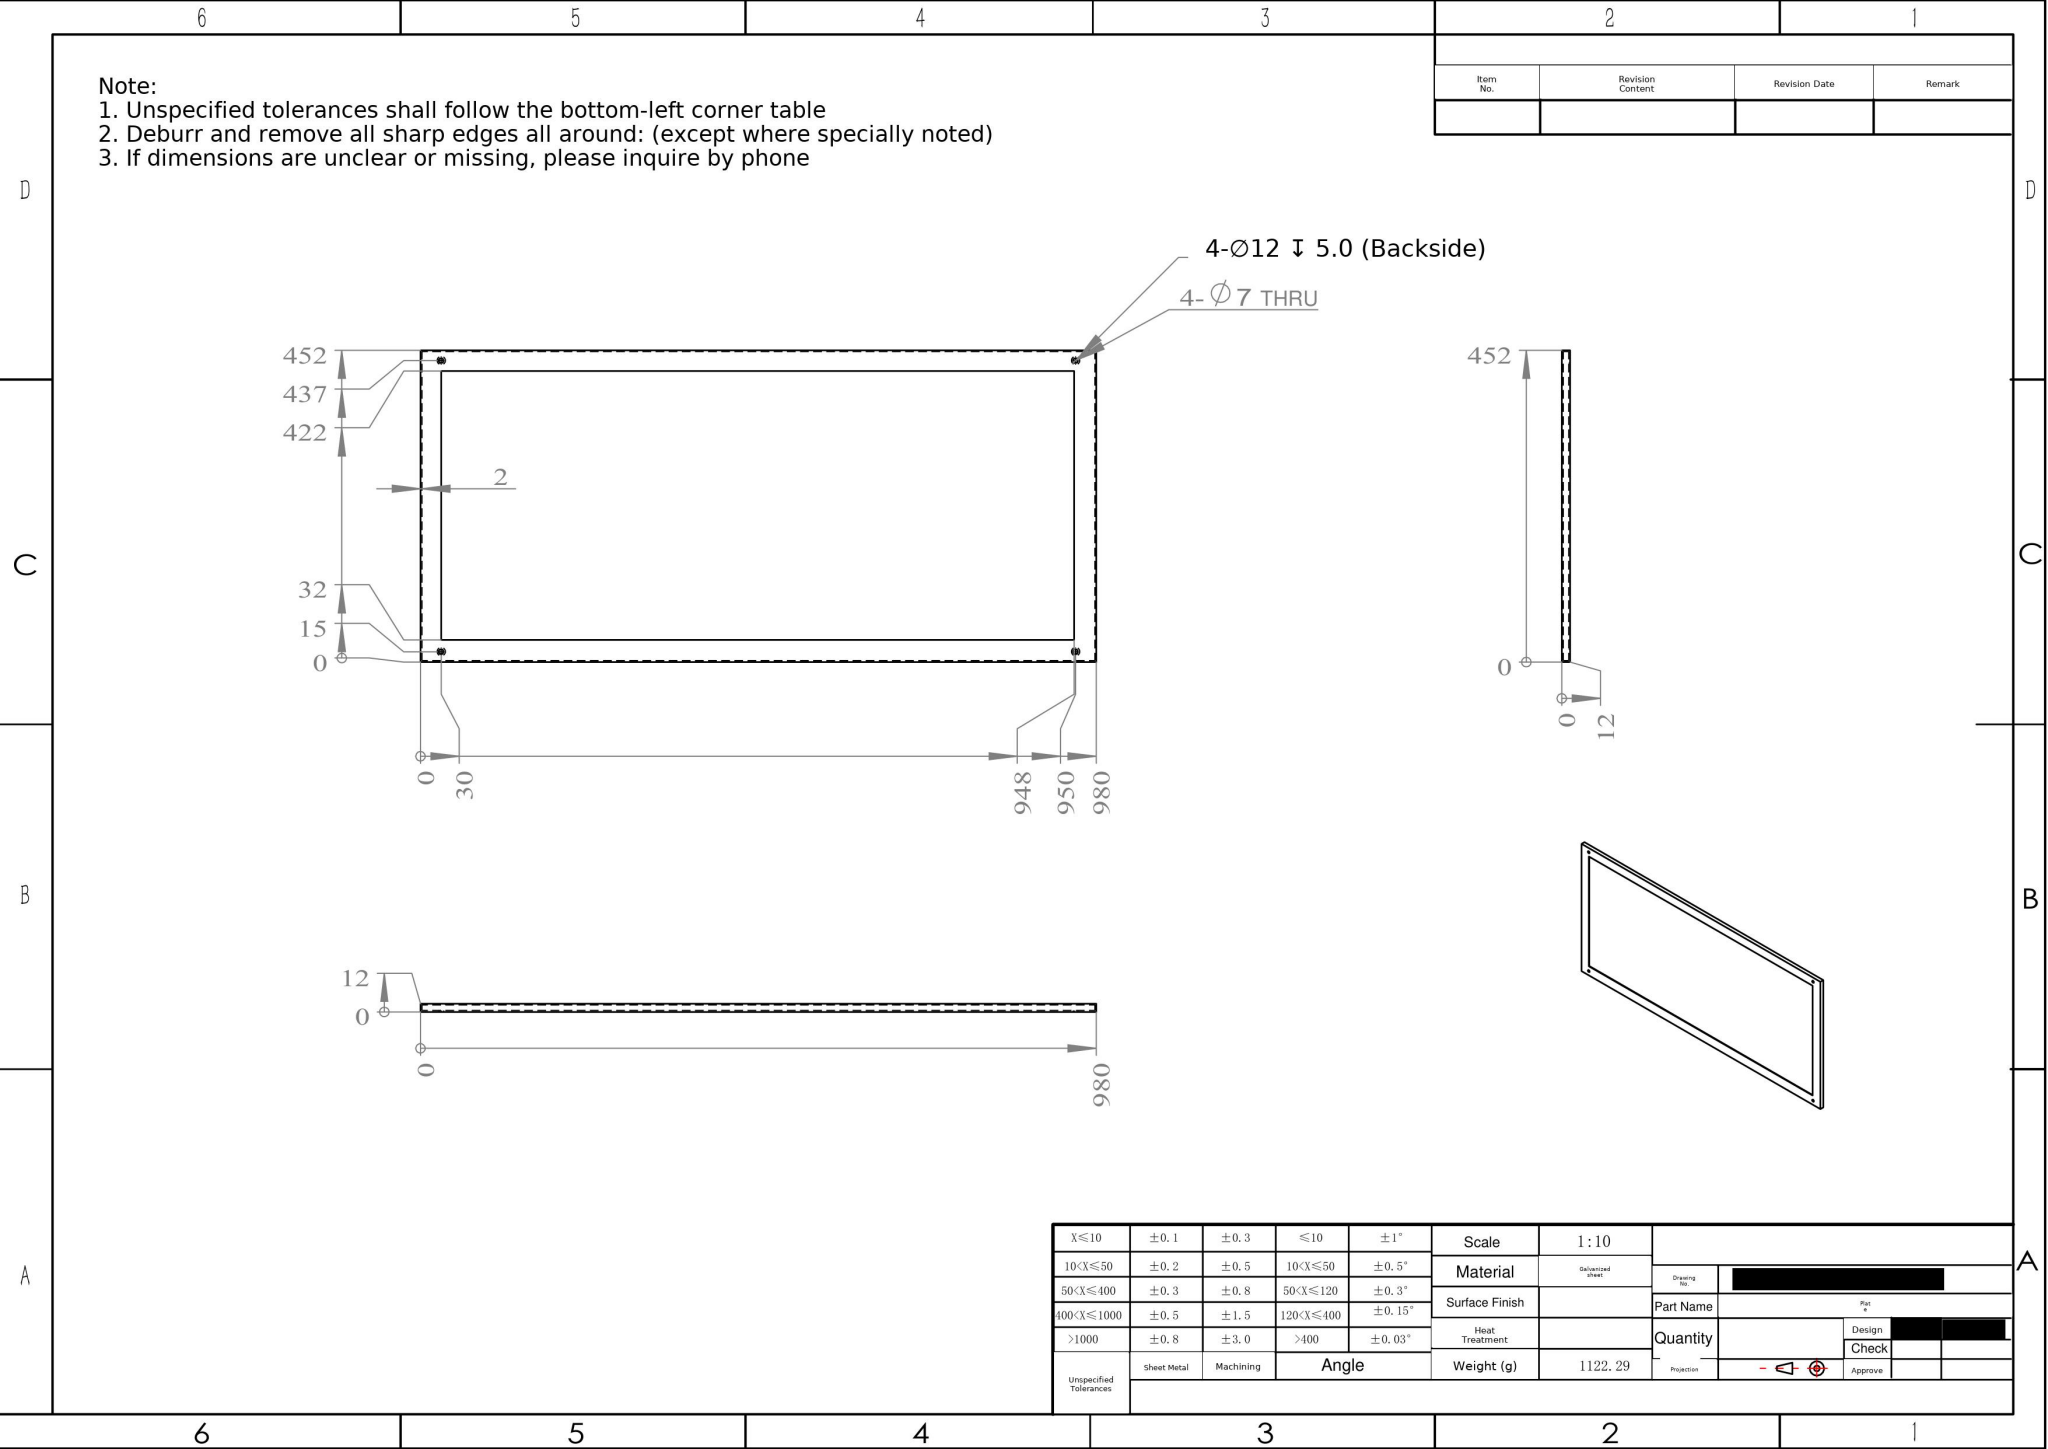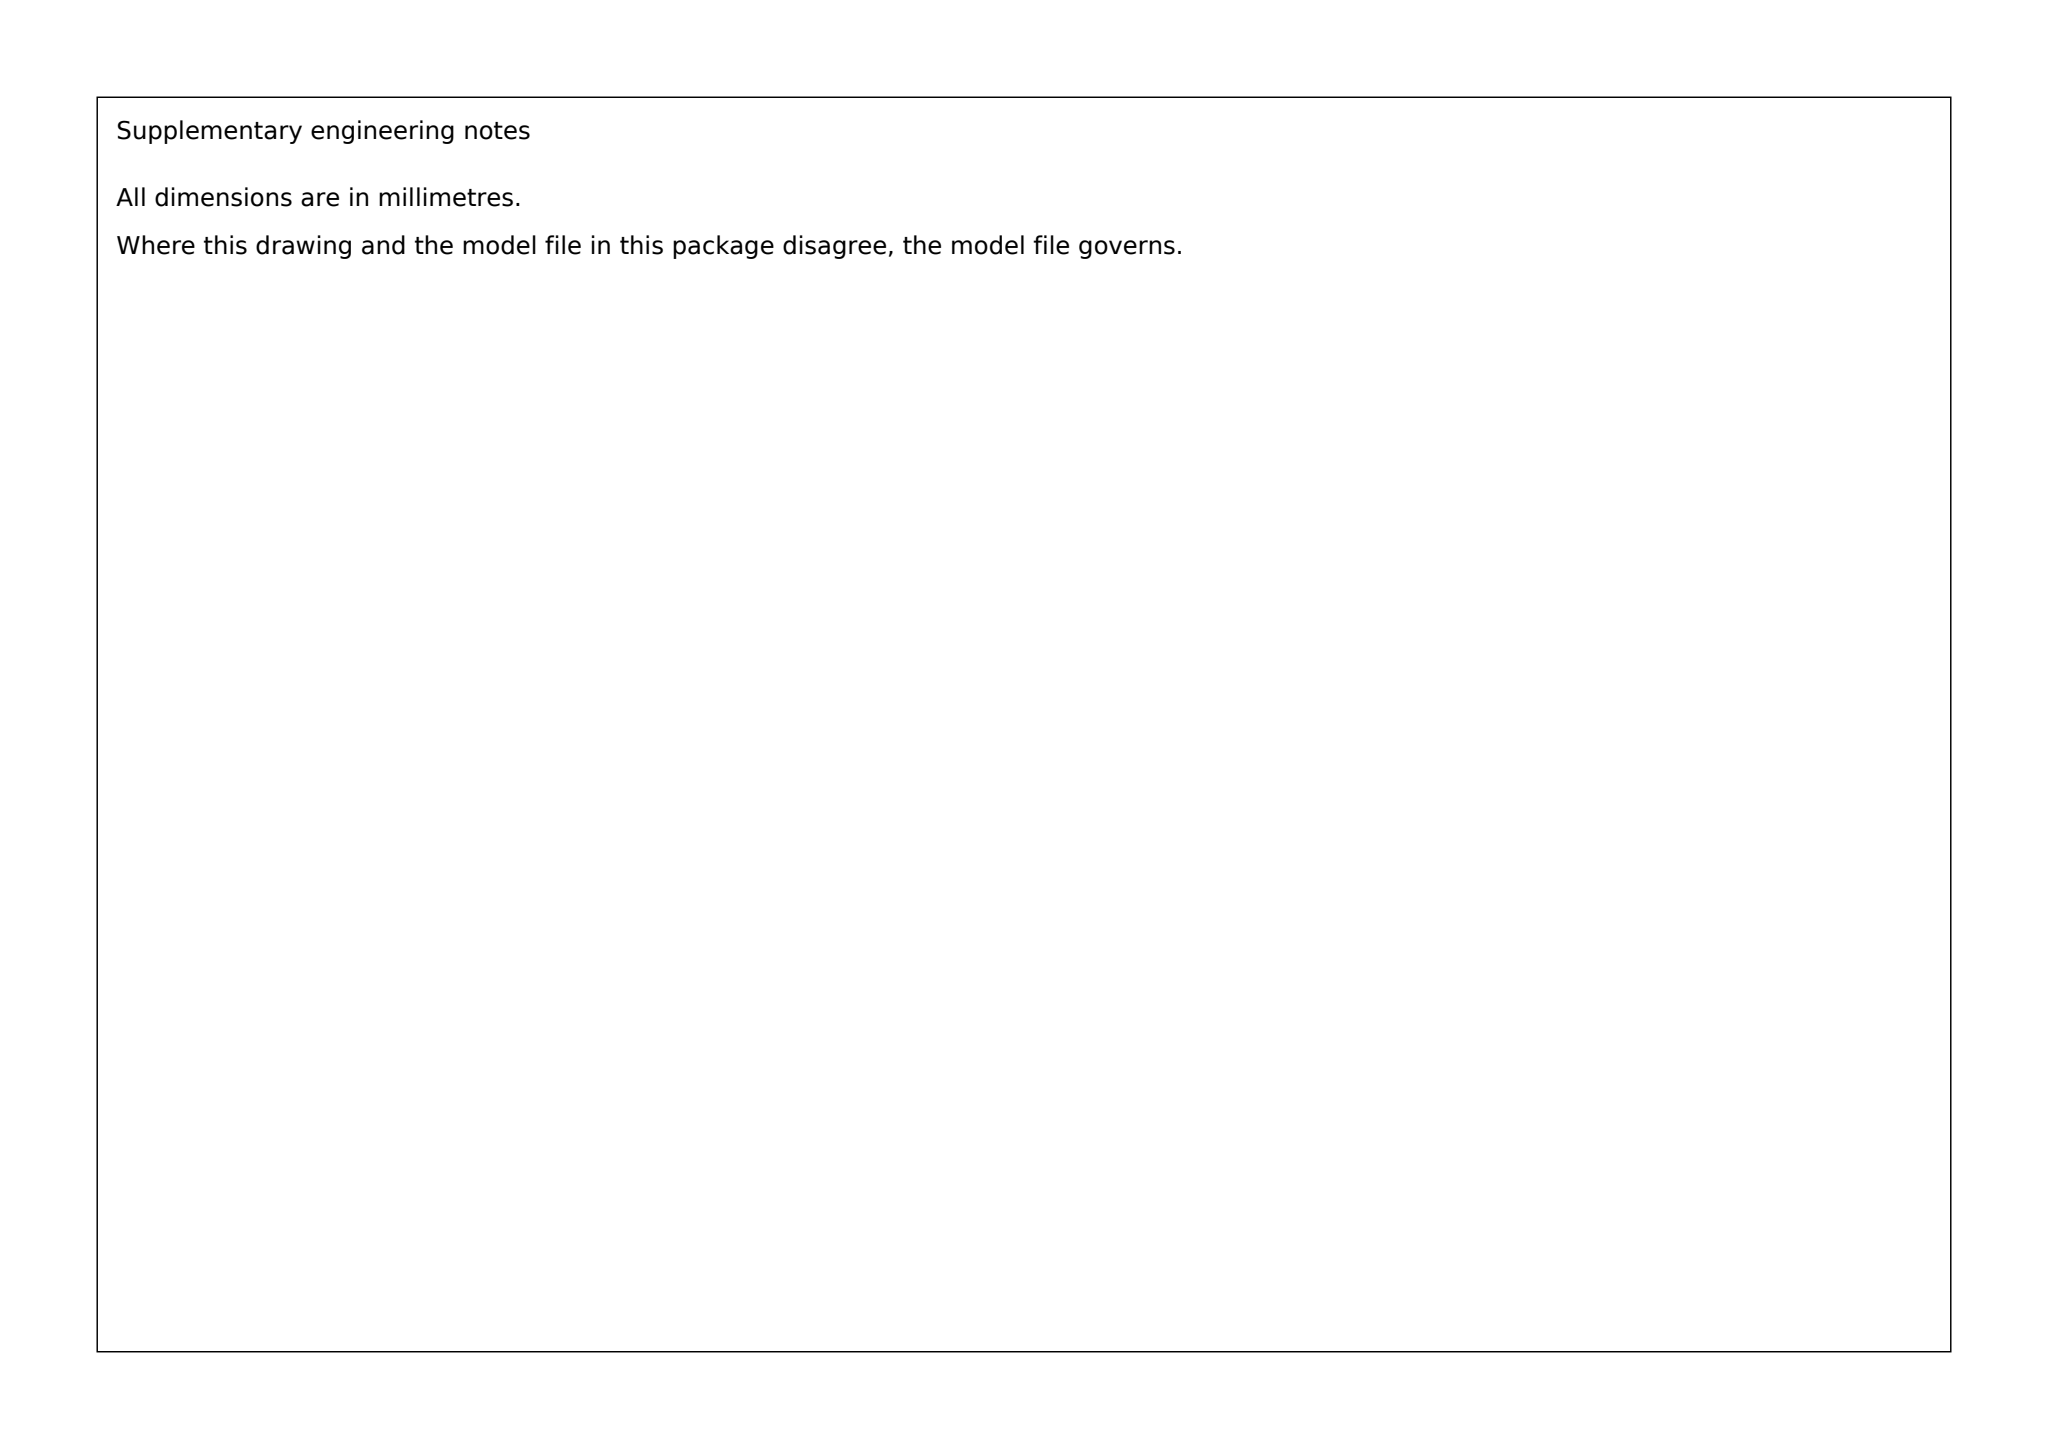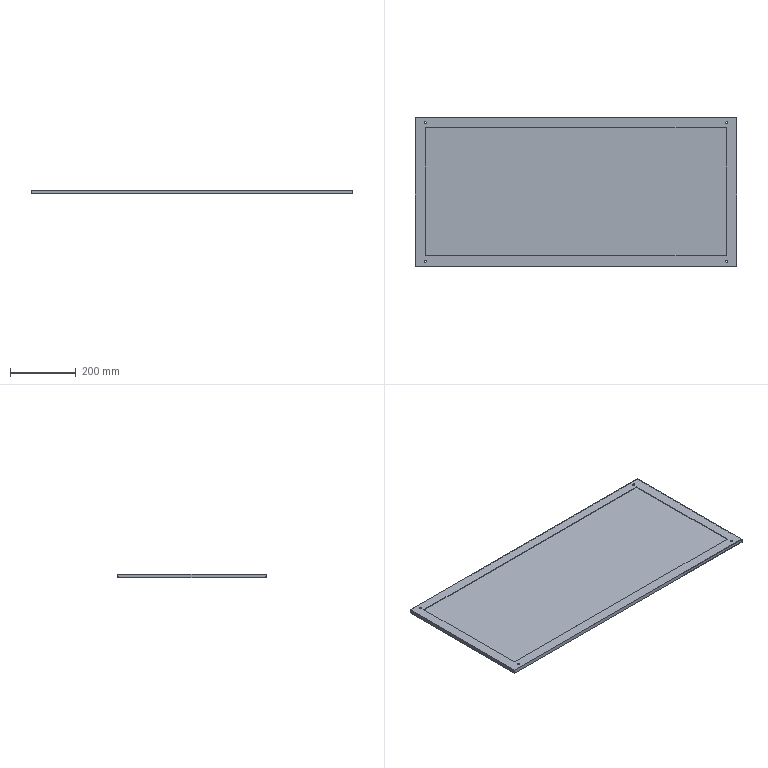Part | SolidWorks | mm | material Galvanized sheet | 1 solid | 32 faces | box 980 x 452 x 12 mm | volume 1100283 mm3 | cylinder 16 | plane 16 | commonest cylinder face diameters 7 x8 12 x8
build123d program:
from build123d import *

# Parameters (mm, degrees)
SKETCH1_W           = 980
SKETCH1_H           = 452
BOSS_EXTRUDE1_DEPTH = 12
SHELL1_T            = -2
SKETCH2_W           = 980
SKETCH2_H           = 452
SKETCH2_W_2         = 918
SKETCH2_H_2         = 390
BOSS_EXTRUDE2_DEPTH = 2
SKETCH3_R           = 6
CUT_EXTRUDE1_DEPTH  = 5
SKETCH4_R           = 3.5
CUT_EXTRUDE2_DEPTH  = 1080.281


with BuildPart() as part:
    # Sketch1 → Boss-Extrude1 (new body)
    with BuildSketch(Plane.XY):
        with Locations((490, -226)):
            Rectangle(SKETCH1_W, SKETCH1_H)
    extrude(amount=BOSS_EXTRUDE1_DEPTH)

    # Shell1
    shell1_openings = [part.faces().sort_by_distance(p)[0] for p in [
        (490, -226, 12),
    ]]
    offset(amount=SHELL1_T, openings=shell1_openings, kind=Kind.INTERSECTION)

    # Sketch2 → Boss-Extrude2 (add)
    with BuildSketch(Plane.XY.offset(12)):
        with Locations((490, -226)):
            Rectangle(SKETCH2_W, SKETCH2_H)
        with Locations((489, -225)):
            Rectangle(SKETCH2_W_2, SKETCH2_H_2, mode=Mode.SUBTRACT)
    extrude(amount=-BOSS_EXTRUDE2_DEPTH)

    # Sketch3 → Cut-Extrude1 (cut)
    with BuildSketch(Plane(origin=(0, 0, 0), x_dir=(-1, 0, 0), z_dir=(0, 0, -1))):
        with Locations((-950, -15)):
            Circle(SKETCH3_R)
        with Locations((-30, -15)):
            Circle(SKETCH3_R)
        with Locations((-950, -437)):
            Circle(SKETCH3_R)
        with Locations((-30, -437)):
            Circle(SKETCH3_R)
    extrude(amount=-CUT_EXTRUDE1_DEPTH, mode=Mode.SUBTRACT)

    # Sketch4 → Cut-Extrude2 (cut, through all)
    with BuildSketch(Plane(origin=(0, 0, 0), x_dir=(-1, 0, 0), z_dir=(0, 0, -1))):
        with Locations((-950, -15)):
            Circle(SKETCH4_R)
        with Locations((-30, -15)):
            Circle(SKETCH4_R)
        with Locations((-30, -437)):
            Circle(SKETCH4_R)
        with Locations((-950, -437)):
            Circle(SKETCH4_R)
    extrude(amount=-CUT_EXTRUDE2_DEPTH, mode=Mode.SUBTRACT)


solid = part.part